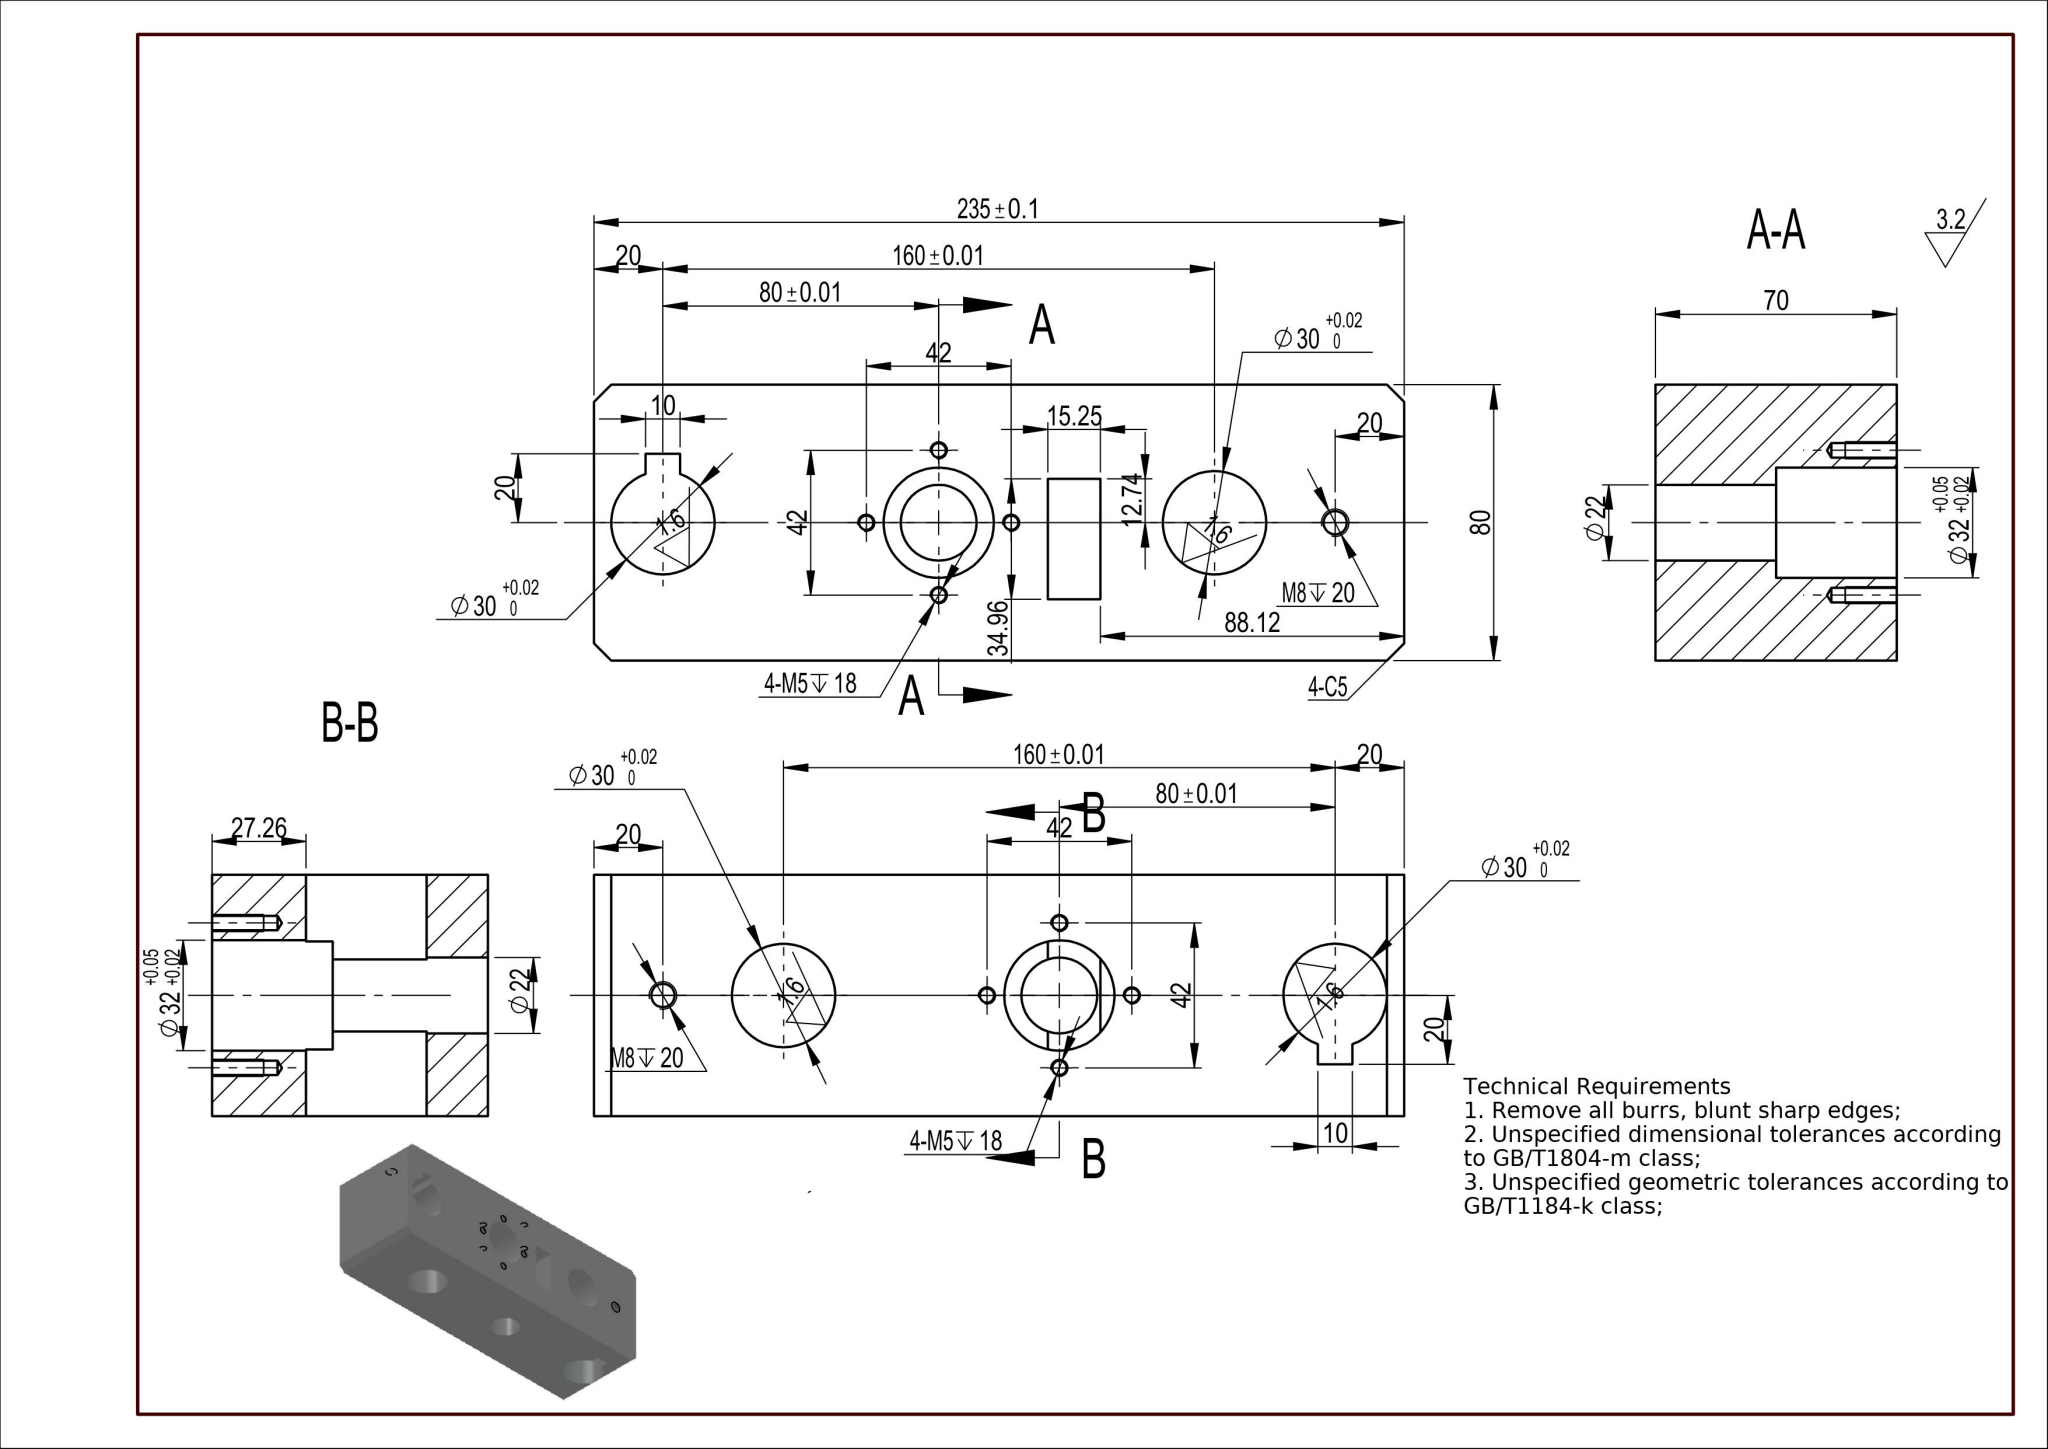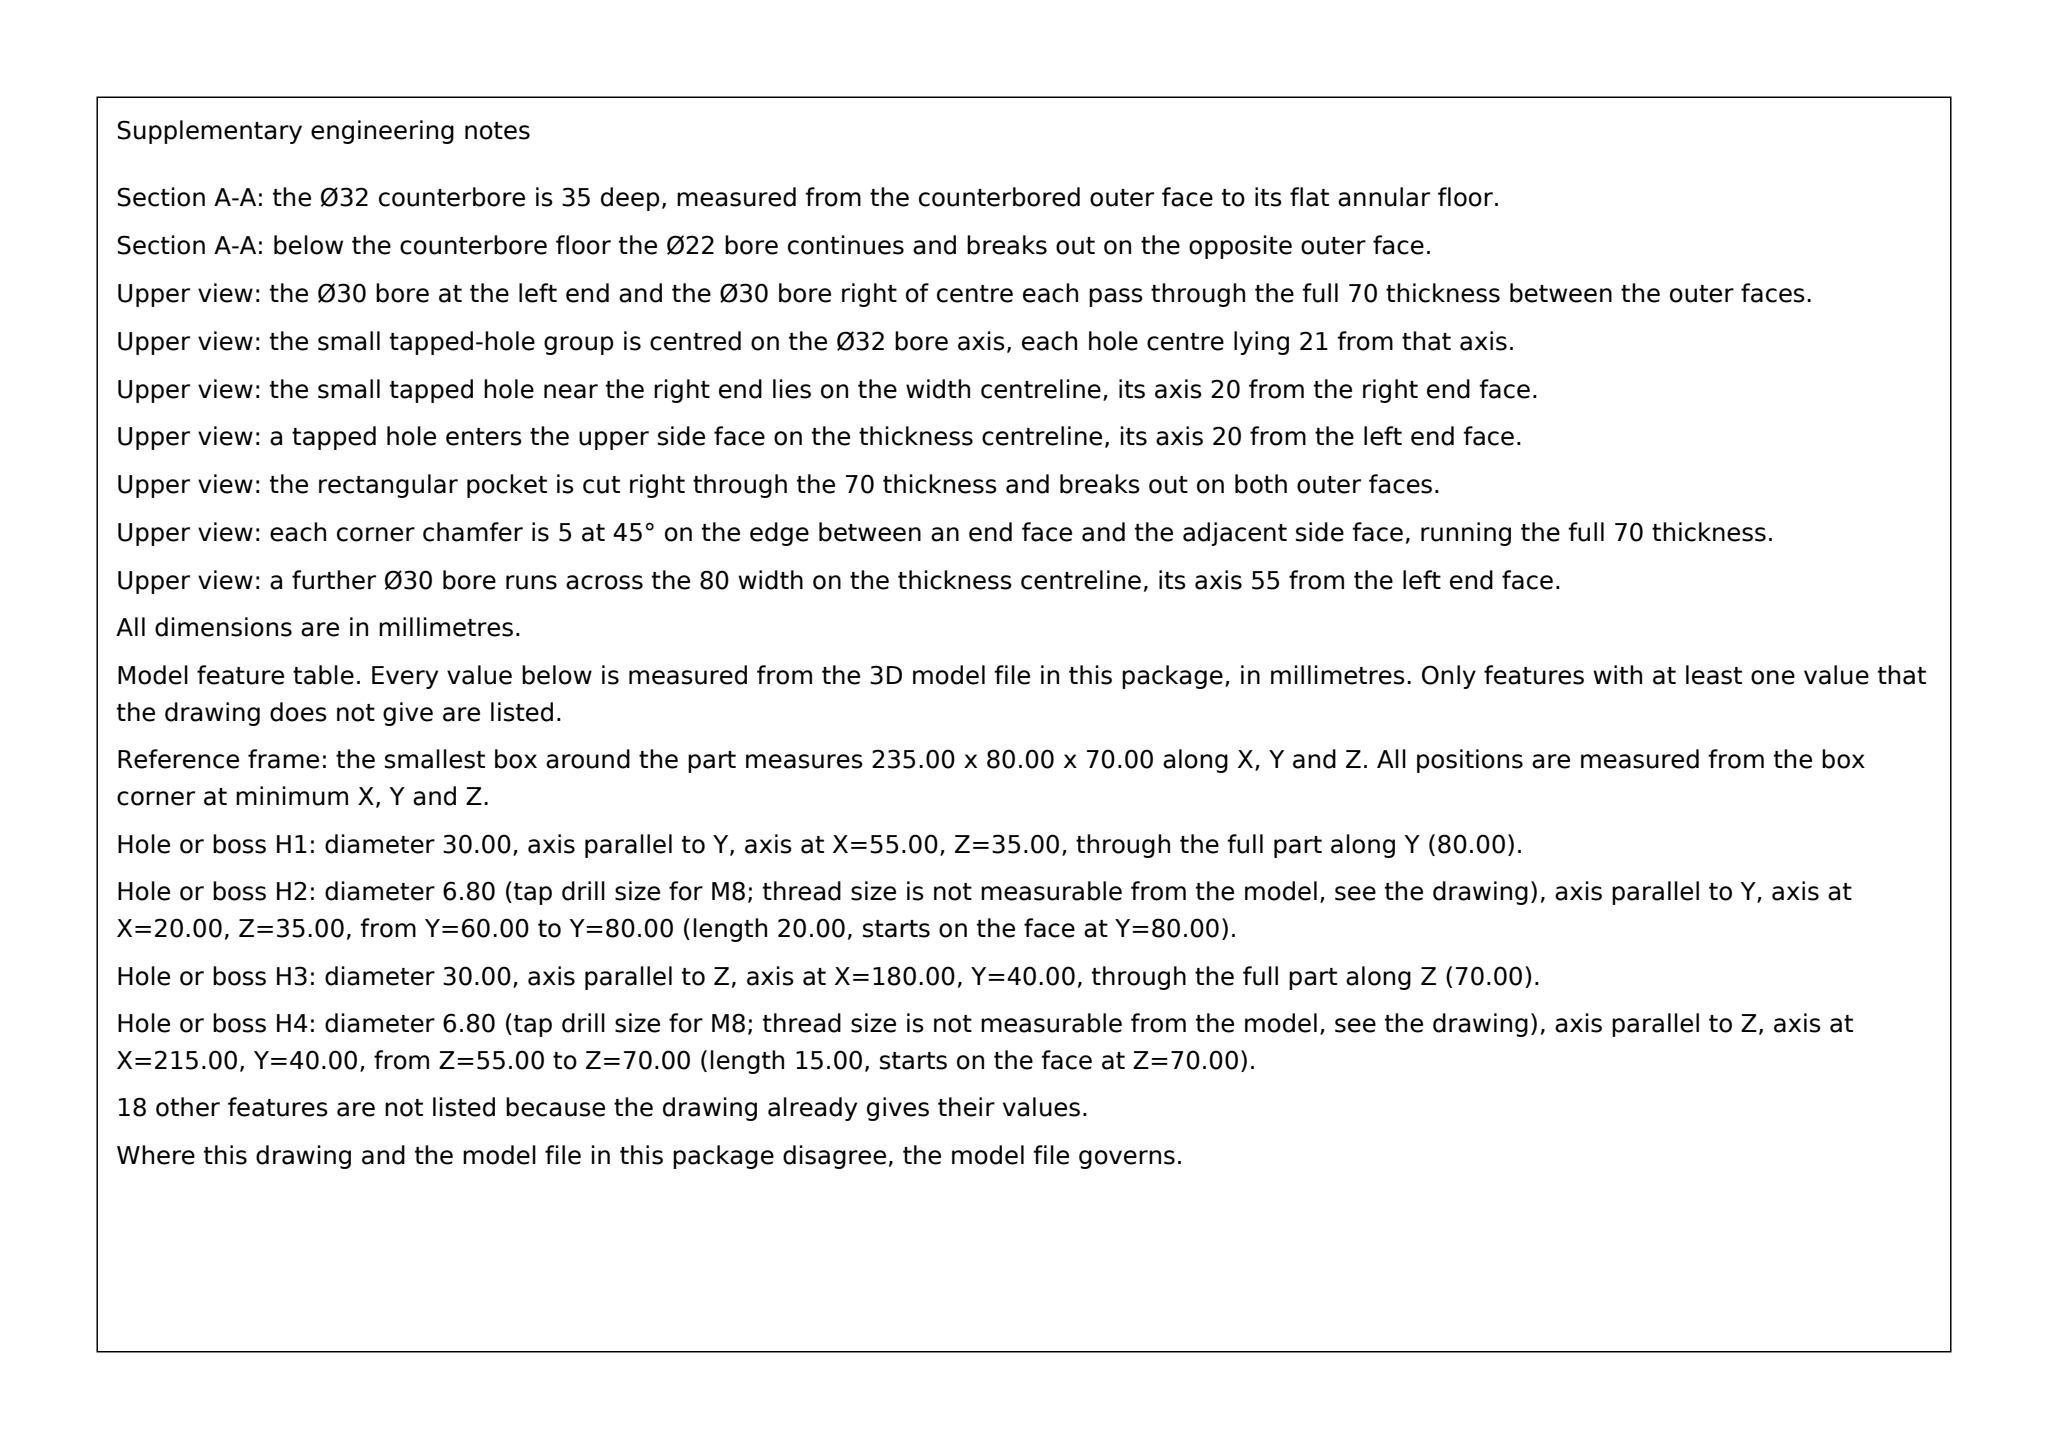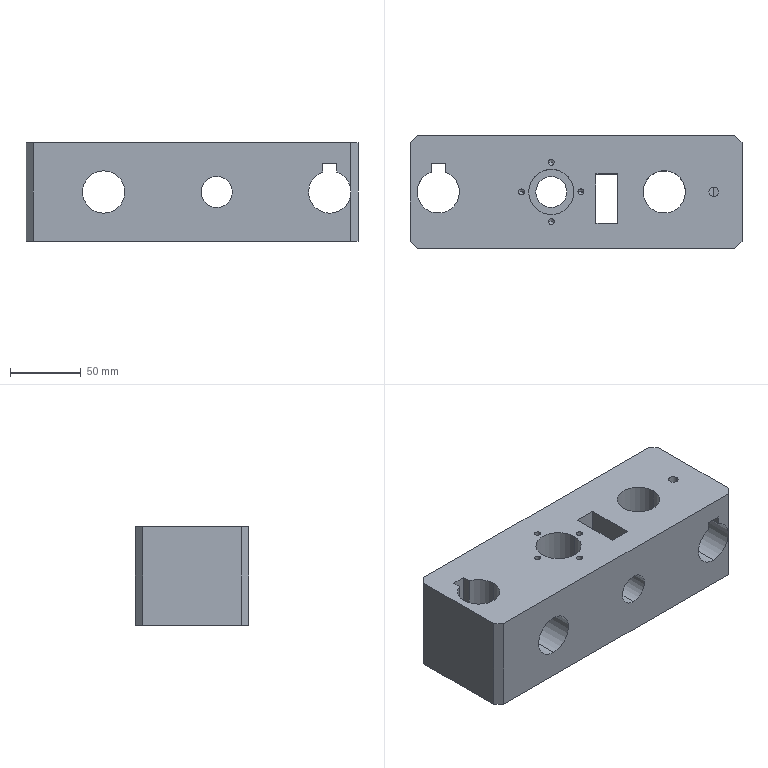Part | SolidWorks | mm | 1 solid | 78 faces | box 235 x 80 x 70 mm | volume 975703 mm3 | cylinder 37 | plane 25 | cone 16 | commonest cylinder face diameters 4.2 x16 30 x9 6.8 x4 32 x4 22 x4
Drawing notes:
RECTANGULAR POCKET 15.25 X 34.96, DEPTH 15 FROM TOP FACE (Z=70); POCKET WALLS AT X=131.63 AND X=146.88 FROM LEFT END, Y=17.78 AND Y=52.74 FROM BOTTOM EDGE | from the solid: axis_planes: x=131.63 & x=146.88 (15.25 wide), y=17.78 & y=52.74 (34.96 wide), floor plane z=55.0 vs top face z=70.0
SECTION A-A BORE AT X=100, Y=40: Ø32 (+0.05/+0.02) DEPTH 35 FROM TOP FACE (Z=70), THEN Ø22 THRU REMAINING 35 TO BOTTOM FACE | from the solid: cylinders: [32, z, (100,40), 35] and [22, z, (100,40), 35]; bbox z extent 70
HORIZONTAL BORE AT X=135, Z=35: Ø32 (+0.05/+0.02) CBORE DEPTH 35 FROM FRONT FACE (Y=0) | from the solid: cylinder dia 32, axis y, pos [135,null,35], length 35
HORIZONTAL BORE AT X=135, Z=35: Ø22 THRU REMAINING 45 FROM Y=35 TO BACK FACE (Y=80) | from the solid: cylinder dia 22, axis y, pos [135,null,35], length 45; bbox Y=80